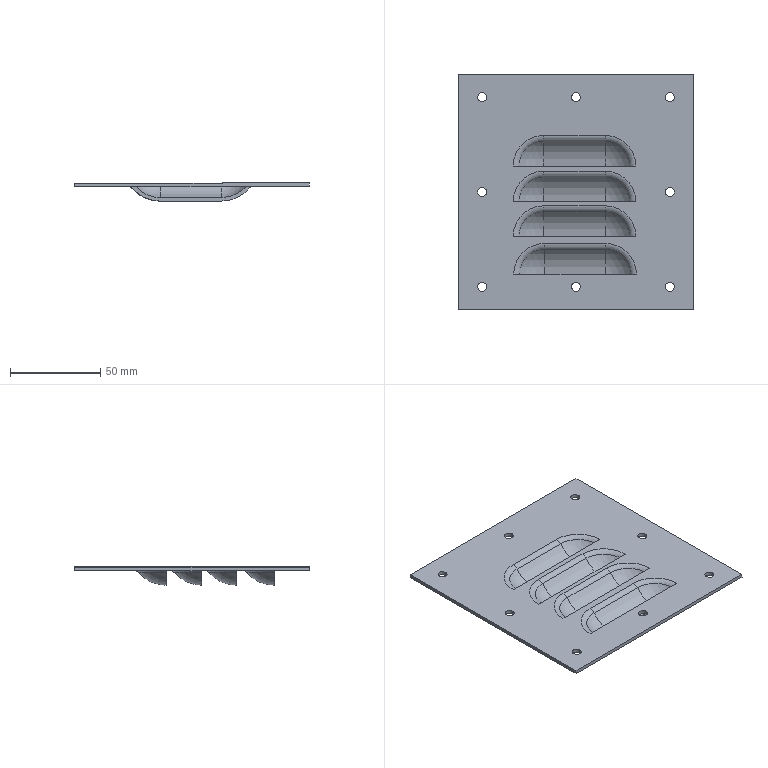Component | SolidWorks | LeftRearDoor-1_Vent-1 | 1 solid | 78 faces | volume 34867 mm3 | cylinder 32 | sphere 16 | torus 16 | plane 14 | commonest cylinder face diameters 5 x16 36 x4 8 x4 4 x4 40 x4 | material AISI 304